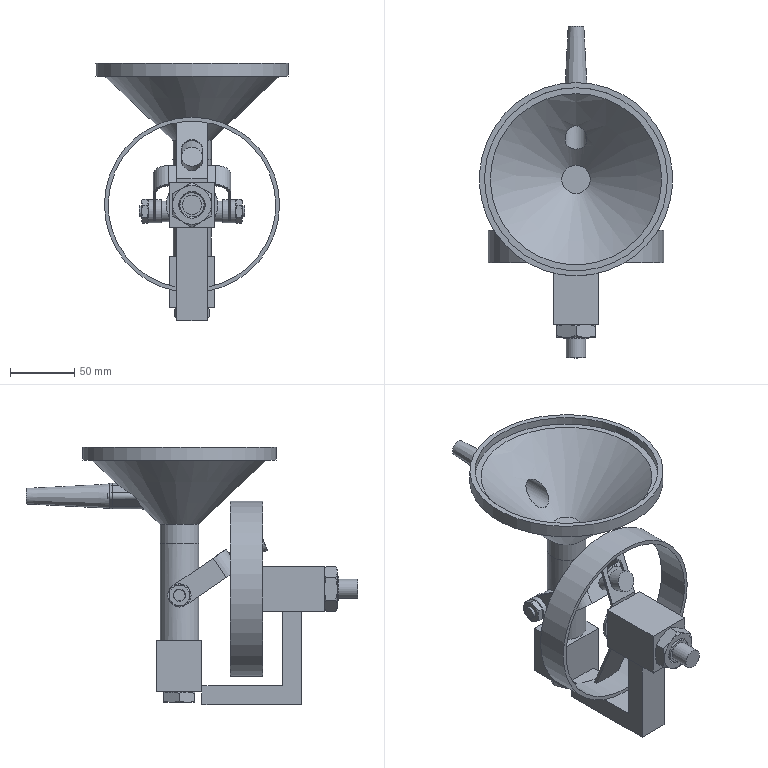Assembly | NX | mm | 13 component files | 14 solids | 287 faces | box 150 x 257.54 x 200 mm | volume 403000 mm3 | plane 143 | cone 78 | cylinder 60 | torus 4 | sphere 2 | commonest cylinder face diameters 20 x8 16 x7 10 x6 6 x4 8.782 x4 22 x3 1.886 x2 3.8 x2
Bill of materials:
unnamed part 1 | 1 |  | Conical funnel-shaped shell with a thin cylindrical rim band at the wide top, a short cylindrical spout at the narrow bottom with a central through-opening, and a small cylindrical side port that sticks out through the cone wall at an angle.
unnamed part 2 | 1 |  | Block-and-bar body: a larger rectangular block with a round through-hole, a vertical rectangular bar running down from it, a horizontal bar running sideways from the bottom of that bar, and a smaller cube-like block at the far end with its own round hole on a different axis. In the front view the outline is a stepped L.
unnamed part 3 | 1 |  | Straight hollow tube that tapers along its length, with a flat diamond-shaped (two-lobe) flange at the wide end. The flange has two small through-holes, one in each lobe, on either side of the central bore.
unnamed part 4 | 1 |  | Bent U-shaped strap (bracket) with a short cylindrical boss at the end of each leg, each with a hole through it, and a ball-ended stud sticking out from the outside of the base of the U.
unnamed part 5 | 1 |  | Cross-shaped shaft body: a central cylinder with stepped, smaller-diameter shaft ends along its main axis, and two stepped cylindrical pins sticking out on opposite sides, perpendicular to the main axis.
GB-T70.1-2000,M2x5 | 2 |  | Hexagon Socket Head Cap Screw, GB-T 70.1-2000,M2x5
unnamed part 6 | 1 |  | Wheel-like body: a thin cylindrical outer ring joined to a central round hub by a single straight bar running across the full diameter, with a stepped shaft coming out of the hub on one side. One half of the bar has a slotted (elongated) through-hole.
GB-T6173-2000,M20x1.5 | 1 |  | Thin hexagonal nut-shaped body: a short hexagonal prism with a large central round through-bore and chamfered corners on both end faces.
GB-T6172_1-2000,M16x2 | 1 |  | Hexagon Thin Nut, Chamfered, GB-T 6172.1-2000,M16x2
GB-T6172_1-2000,M10x1.5 | 2 |  | Hexagon Thin Nut, Chamfered, GB-T 6172.1-2000,M10x1.5
unnamed part 7 | 1 |  | Solid flanged cylinder (plug or bushing-like shape): a straight cylindrical body with a thin, larger-diameter round flange at one end.
Mates:
1. fix | 6 1 component
2. concentric | 2 1 edge | 6 1 edge
3. concentric | 1 1 edge | 2 1 edge
4. touch align | 3 1 face | 2 1 face
5. center | 3 1 face | 3 1 face | 2 1 face | 2 1 face
6. touch align | 5 1 face | 6 1 face
7. concentric | GB-T6173-2000_M20x1_5 1 edge | 6 1 edge
8. concentric | GB-T6172_1-2000_M16x2 1 edge | 6 1 edge
9. concentric | GB-T6172_1-2000_M10x1_5 1 edge | 3 1 edge
10. concentric | GB-T6172_1-2000_M10x1_5 2 edge | 3 1 edge
11. touch align | 7 1 face | 1 1 face
12. concentric | 7 1 edge | 1 1 edge
13. concentric | GB-T70_1-2000_M2x5 2 edge | 7 1 edge
14. concentric | GB-T70_1-2000_M2x5 1 edge | 7 1 edge
15. touch align | 4 1 face | 3 1 face
16. touch align | 5 1 face | 4 1 face